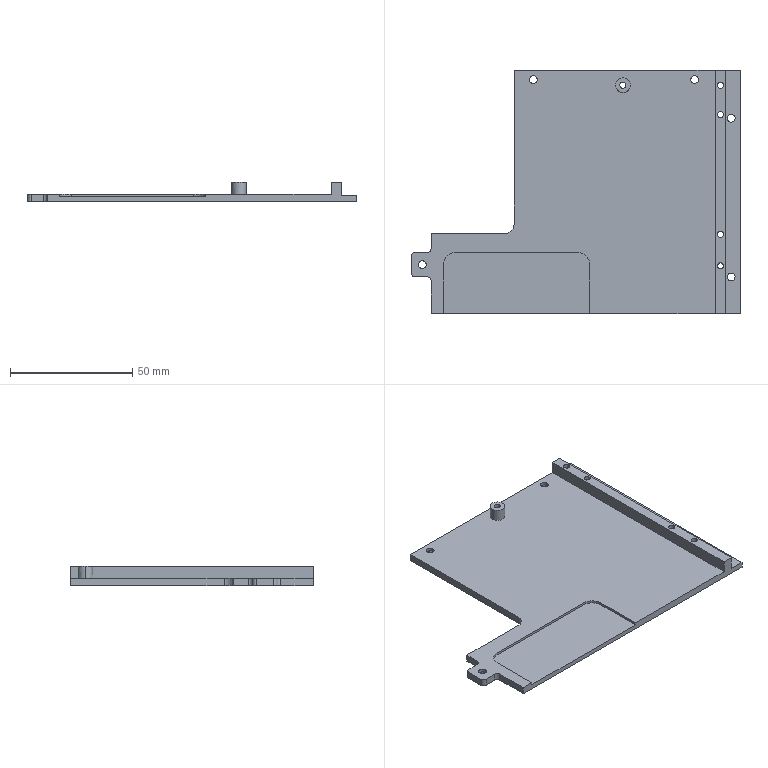CAM job | Mastercam | mm | 17 operations | part box 134.7 x 99.55 x 8
1. Contour (Ramp) | 8 - 8C
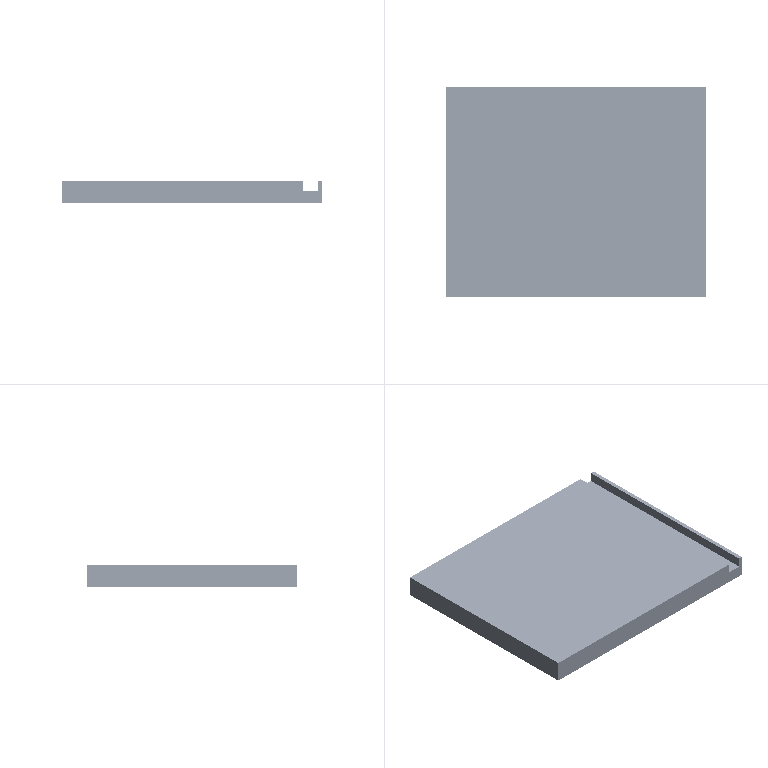2. Pocket (Standard) | 8 - 8C
3. Contour (Ramp) | 8 - 8C
4. Pocket (Standard) | 9 - 8J
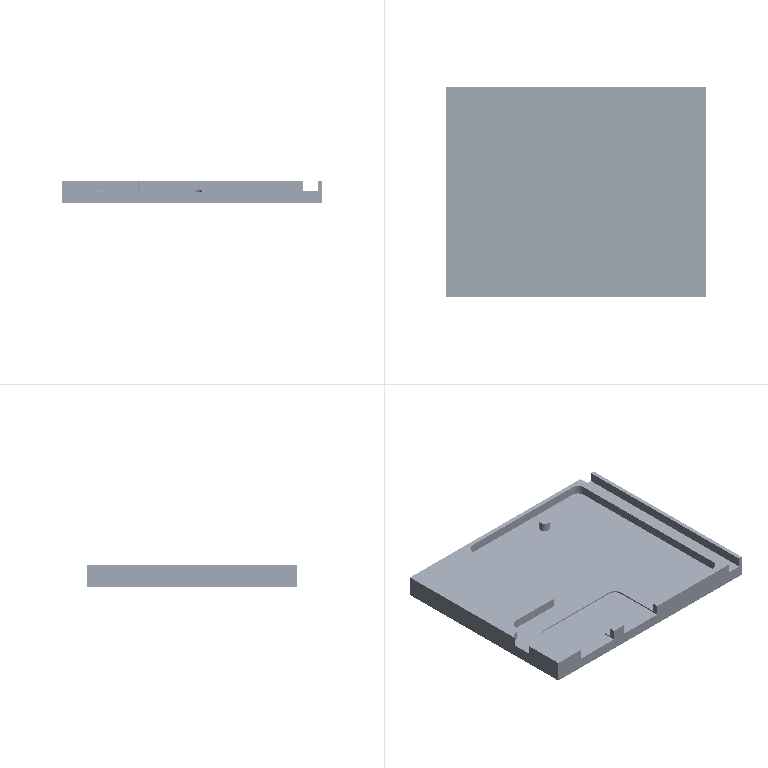5. Contour (2D) | 9 - 8J
6. Contour (2D) | 9 - 8J
7. Contour (Ramp) | 8 - 8C
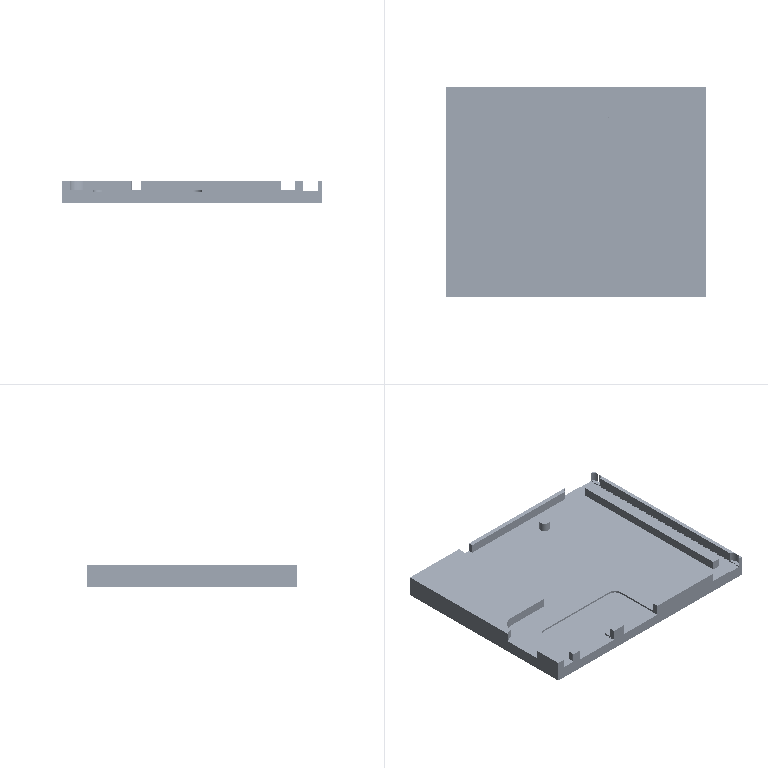8. Contour (Ramp) | 8 - 8C
9. Contour (2D) | 9 - 8J
10. Contour (Remachining) | 13 - 3J
11. Drill/Counterbore | 1 - 4 倒角刀
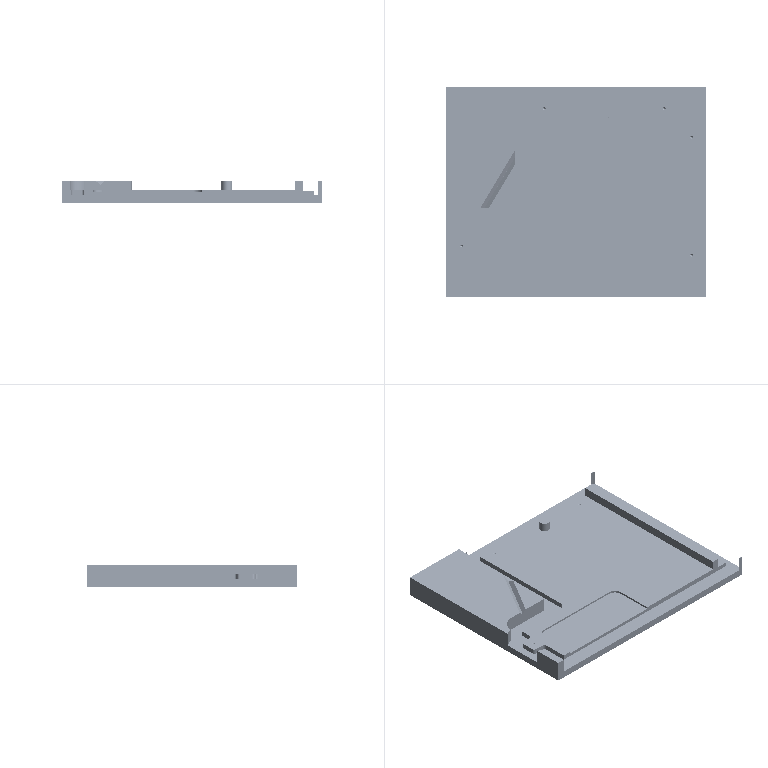12. Drill/Counterbore | 1 - 4 倒角刀
13. Peck Drill | 21 - 3.2 钻头
14. Peck Drill | 7 - 2.5 钻头
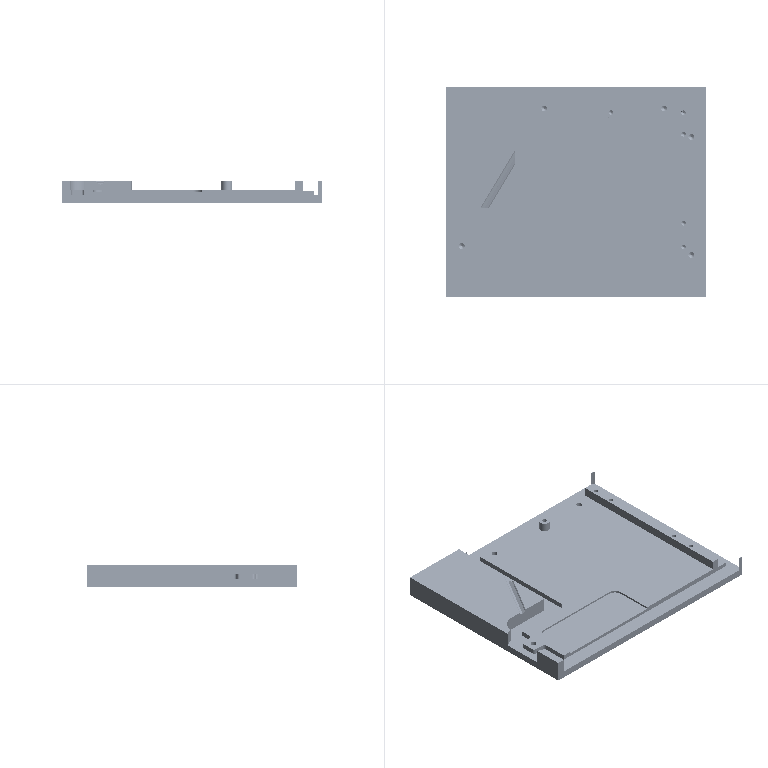15. Chamfer Drill | 1 - 4 倒角刀
16. Chamfer Drill | 1 - 4 倒角刀
17. Model Chamfer | 1 - 4 倒角刀